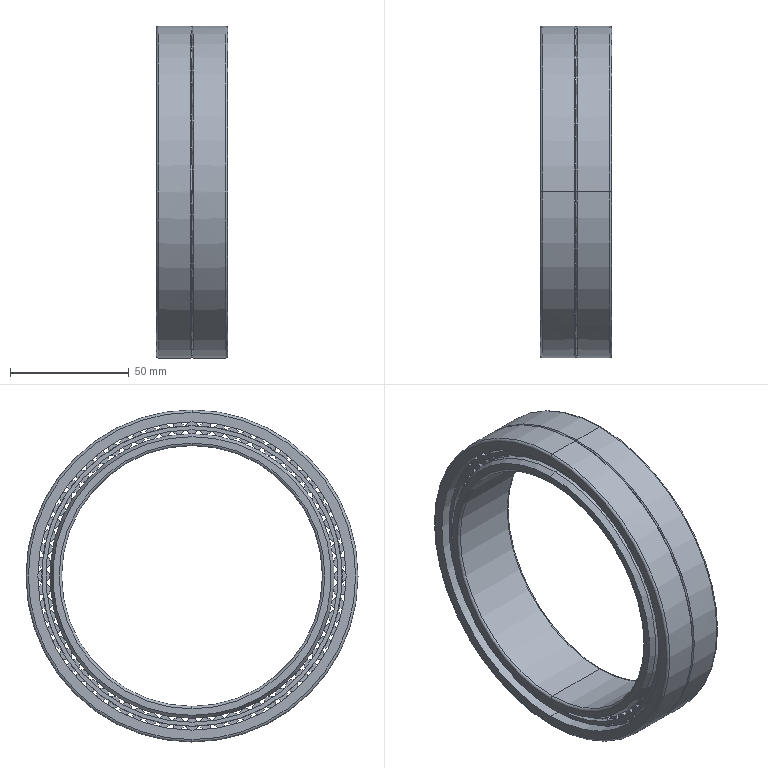Component | SolidWorks | needle roller bearings lm series gb-1 | 3 solids | 472 faces | box 30 x 140 x 140 mm | volume 140008 mm3 | plane 284 | cylinder 166 | torus 18 | cone 4 | commonest cylinder face diameters 5.04 x136 1.5 x8 130 x4 140 x4 120 x4 132 x2 110 x2 119.96 x2
build123d program:
from build123d import *

# Parameters (mm, degrees)
SKETCH2_W               = 20
SKETCH2_H               = 2.52
CIRCULAR_PATTERN1_COUNT = 68
SKETCH4_W               = 25
SKETCH4_H               = 1.68
SKETCH5_R               = 0.5
SKETCH6_R               = 0.75
CUT_EXTRUDE1_DEPTH      = 5


with BuildPart() as part:
    # Sketch1 → Revolve1 (revolve)
    with BuildSketch(Plane.XY, mode=Mode.PRIVATE) as revolve1_sk:
        with BuildLine():
            Line((10, 65.02), (10, 65))
            Line((10, 65), (15, 65))
            Line((15, 65), (15, 69))
            ThreePointArc((15, 69), (14.707, 69.707), (14, 70))
            Line((14, 70), (-14, 70))
            ThreePointArc((-14, 70), (-14.707, 69.707), (-15, 69))
            Line((-15, 69), (-15, 65))
            Line((-15, 65), (-10, 65))
            Line((-10, 65), (-10, 65.02))
            Line((-10, 65.02), (10, 65.02))
        make_face()
    revolve(revolve1_sk.sketch.rotate(Axis((-15, 0, 0), (1, 0, 0)), 90), axis=Axis((-15, 0, 0), (1, 0, 0)))

    # Sketch7 → Cut-Revolve2 (revolve, cut)
    with BuildSketch(Plane.XY, mode=Mode.PRIVATE) as cut_revolve2_sk:
        with BuildLine():
            Line((-9.833, 66), (9.833, 66))
            ThreePointArc((9.833, 66), (10.118, 66.118), (10, 65.833))
            Line((10, 65.833), (10, 64.8))
            Line((10, 64.8), (-10, 64.8))
            Line((-10, 64.8), (-10, 65.833))
            ThreePointArc((-10, 65.833), (-10.118, 66.118), (-9.833, 66))
        make_face()
    revolve(cut_revolve2_sk.sketch.rotate(Axis((0, 0, 0), (1, 0, 0)), 90), axis=Axis((0, 0, 0), (1, 0, 0)), mode=Mode.SUBTRACT)

    # Sketch5 → Cut-Revolve1 (revolve, cut)
    with BuildSketch(Plane(origin=(0, 0, 0), x_dir=(1, 0, 0), z_dir=(0, 1, 0)), mode=Mode.PRIVATE) as cut_revolve1_sk:
        with Locations((0, 70)):
            Circle(SKETCH5_R)
    revolve(cut_revolve1_sk.sketch.rotate(Axis((-3.429, 0, 0), (1, 0, 0)), 180), axis=Axis((-3.429, 0, 0), (1, 0, 0)), mode=Mode.SUBTRACT)


with BuildPart() as body_2:
    # Sketch2 → Revolve2 (revolve)
    with BuildSketch(Plane.XY, mode=Mode.PRIVATE) as revolve2_sk:
        with Locations((0, 63.76)):
            Rectangle(SKETCH2_W, SKETCH2_H)
    revolve(revolve2_sk.sketch.rotate(Axis((-21.372, 62.5, 0), (1, 0, 0)), 90), axis=Axis((-21.372, 62.5, 0), (1, 0, 0)))

    # Circular-Pattern1: body 2 ×68 about axis
    circular_pattern1_axis = Axis((0, 0, 0), (1, 0, 0))


with BuildPart() as body_3:
    # Sketch1_4 → Revolve3 (revolve)
    with BuildSketch(Plane.XY, mode=Mode.PRIVATE) as revolve3_sk:
        with BuildLine():
            ThreePointArc((-15, 56), (-14.707, 55.293), (-14, 55))
            Line((-14, 55), (14, 55))
            ThreePointArc((14, 55), (14.707, 55.293), (15, 56))
            Line((15, 56), (15, 58.75))
            Line((15, 58.75), (12.5, 60))
            Line((12.5, 60), (10, 60))
            Line((10, 60), (10, 59.98))
            Line((10, 59.98), (-10, 59.98))
            Line((-10, 59.98), (-10, 60))
            Line((-10, 60), (-12.5, 60))
            Line((-12.5, 60), (-15, 58.75))
            Line((-15, 58.75), (-15, 56))
        make_face()
    revolve(revolve3_sk.sketch.rotate(Axis((-15, 0, 0), (1, 0, 0)), 90), axis=Axis((-15, 0, 0), (1, 0, 0)))


with BuildPart() as body_2_1:
    add(body_2.part)
    for i in range(1, CIRCULAR_PATTERN1_COUNT):
        add(body_2.part.rotate(circular_pattern1_axis, i * 360 / CIRCULAR_PATTERN1_COUNT))

    # Sketch4 → Revolve4 (revolve)
    with BuildSketch(Plane.XY, mode=Mode.PRIVATE) as revolve4_sk:
        with Locations((0, 62.5)):
            Rectangle(SKETCH4_W, SKETCH4_H)
    revolve(revolve4_sk.sketch.rotate(Axis((-15, 0, 0), (1, 0, 0)), 90), axis=Axis((-15, 0, 0), (1, 0, 0)))


with BuildPart() as cut_extrude1_tool:
    # Sketch6 → Cut-Extrude1 (new body)
    with BuildSketch(Plane(origin=(0, 70, 0), x_dir=(1, 0, 0), z_dir=(0, 1, 0))):
        with Locations(Location((0, 0, 0), (0, 0, 270))):
            Circle(SKETCH6_R)
    cut_extrude1 = extrude(amount=-CUT_EXTRUDE1_DEPTH)


with BuildPart() as part_1:
    add(part.part)

    # Cut-Extrude1: cut by cut_extrude1_tool
    add(cut_extrude1_tool.part, mode=Mode.SUBTRACT)


with BuildPart() as body_2_2:
    add(body_2_1.part)

    # Cut-Extrude1: cut by cut_extrude1_tool
    add(cut_extrude1_tool.part, mode=Mode.SUBTRACT)


with BuildPart() as mirror1_tool:
    # Mirror1: Cut-Extrude1 across plane
    add(cut_extrude1.mirror(Plane.ZX))


with BuildPart() as part_2:
    add(part_1.part)

    # Mirror1: cut by mirror1_tool
    add(mirror1_tool.part, mode=Mode.SUBTRACT)


with BuildPart() as body_2_3:
    add(body_2_2.part)

    # Mirror1: cut by mirror1_tool
    add(mirror1_tool.part, mode=Mode.SUBTRACT)


solid = Compound([body_3.part, part_2.part, body_2_3.part])

# Placed as in the assembly
solid = solid.moved(Location((182.562, 15.116, 349), (0, 0, 0)))